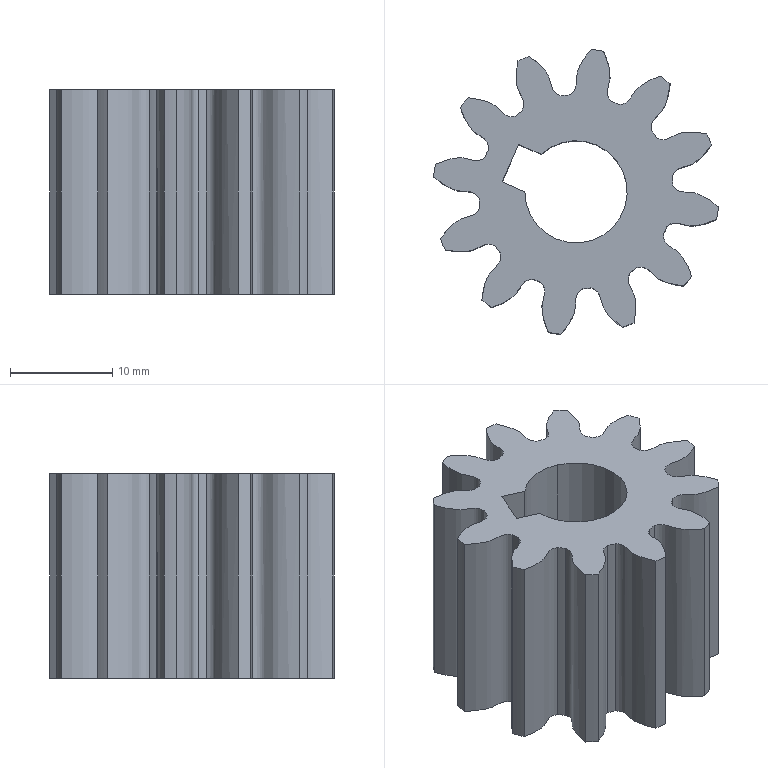Component | SolidWorks | CylindricalGear12x2Small-1 | 1 solid | 56 faces | volume 7015 mm3 | cylinder 27 | spline 24 | plane 5 | commonest cylinder face diameters 28 x12 19 x12 10 x3